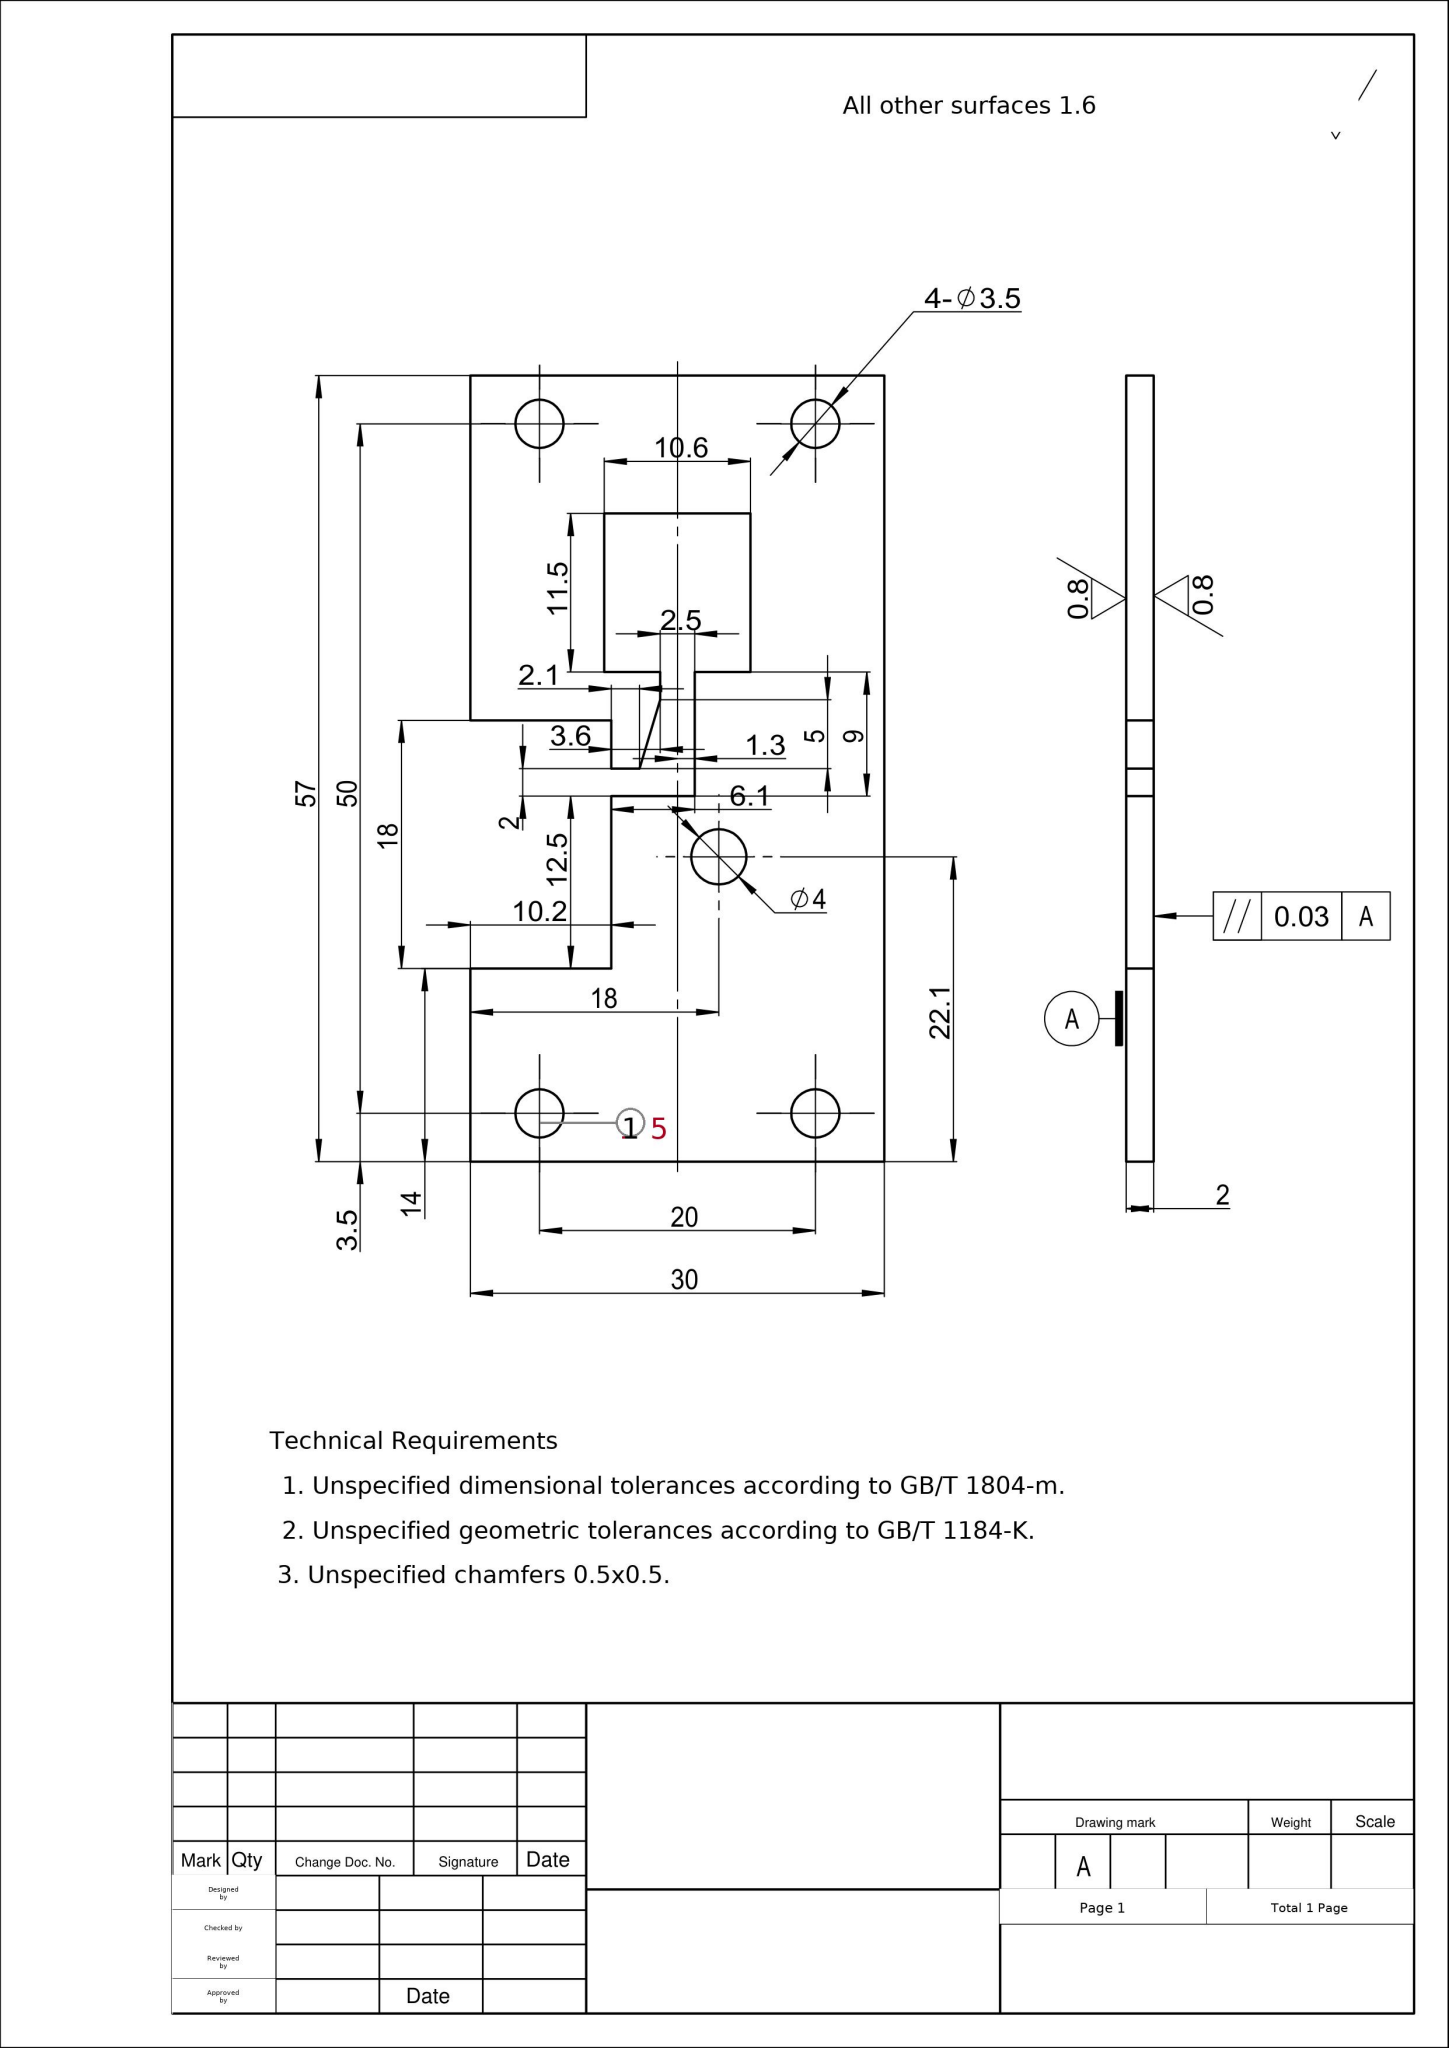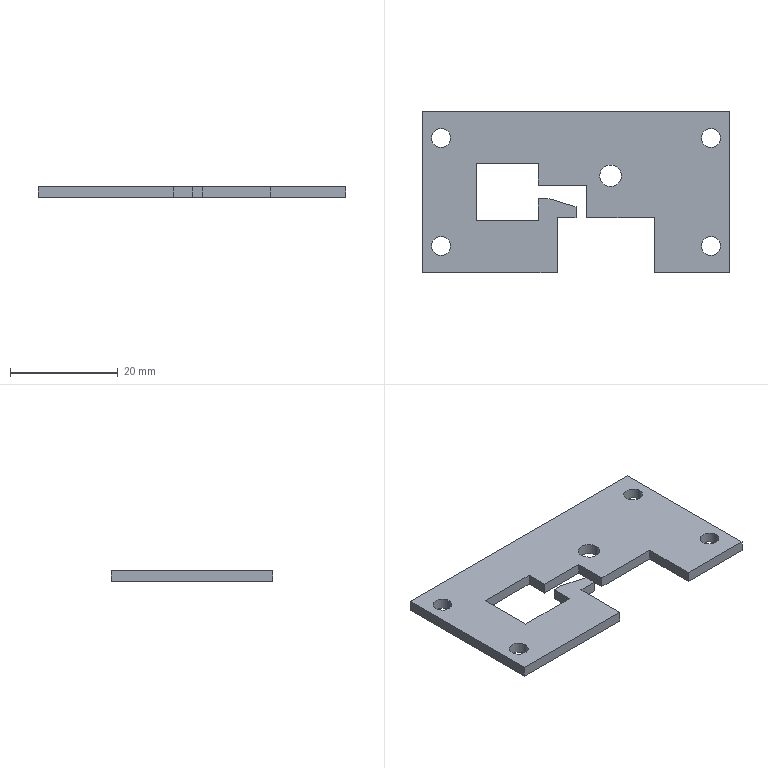Part | SolidWorks | mm | 1 solid | 31 faces | box 57 x 30 x 2 mm | volume 2640 mm3 | plane 21 | cylinder 10 | commonest cylinder face diameters 3.5 x8 4 x2
STEP:
#1=CARTESIAN_POINT('',(32.9,-12.,0.));
#2=VERTEX_POINT('',#1);
#3=CARTESIAN_POINT('',(36.9,-12.,0.));
#4=VERTEX_POINT('',#3);
#5=CARTESIAN_POINT('',(34.9,-12.,0.));
#6=DIRECTION('',(0.,0.,1.));
#7=DIRECTION('',(1.,0.,0.));
#8=AXIS2_PLACEMENT_3D('',#5,#6,#7);
#9=CIRCLE('',#8,2.);
#10=EDGE_CURVE('',#2,#4,#9,.T.);
#11=ORIENTED_EDGE('',*,*,#10,.F.);
#12=CARTESIAN_POINT('',(32.9,-12.,2.));
#13=VERTEX_POINT('',#12);
#14=CARTESIAN_POINT('',(32.9,-12.,0.));
#15=DIRECTION('',(0.,0.,1.));
#16=VECTOR('',#15,1000.);
#17=LINE('',#14,#16);
#18=EDGE_CURVE('',#2,#13,#17,.T.);
#19=ORIENTED_EDGE('',*,*,#18,.T.);
#20=CARTESIAN_POINT('',(36.9,-12.,2.));
#21=VERTEX_POINT('',#20);
#22=CARTESIAN_POINT('',(34.9,-12.,2.));
#23=DIRECTION('',(0.,0.,1.));
#24=DIRECTION('',(1.,0.,0.));
#25=AXIS2_PLACEMENT_3D('',#22,#23,#24);
#26=CIRCLE('',#25,2.);
#27=EDGE_CURVE('',#13,#21,#26,.T.);
#28=ORIENTED_EDGE('',*,*,#27,.T.);
#29=CARTESIAN_POINT('',(36.9,-12.,0.));
#30=DIRECTION('',(0.,0.,1.));
#31=VECTOR('',#30,1000.);
#32=LINE('',#29,#31);
#33=EDGE_CURVE('',#4,#21,#32,.T.);
#34=ORIENTED_EDGE('',*,*,#33,.F.);
#35=EDGE_LOOP('',(#11,#19,#28,#34));
#36=FACE_OUTER_BOUND('',#35,.T.);
#37=CARTESIAN_POINT('',(34.9,-12.,0.));
#38=DIRECTION('',(0.,0.,1.));
#39=DIRECTION('',(1.,0.,0.));
#40=AXIS2_PLACEMENT_3D('',#37,#38,#39);
#41=CYLINDRICAL_SURFACE('',#40,2.);
#42=ADVANCED_FACE('',(#36),#41,.F.);
#43=CARTESIAN_POINT('',(5.25,-25.,0.));
#44=VERTEX_POINT('',#43);
#45=CARTESIAN_POINT('',(1.75,-25.,0.));
#46=VERTEX_POINT('',#45);
#47=CARTESIAN_POINT('',(3.5,-25.,0.));
#48=DIRECTION('',(0.,0.,-1.));
#49=DIRECTION('',(1.,0.,0.));
#50=AXIS2_PLACEMENT_3D('',#47,#48,#49);
#51=CIRCLE('',#50,1.75);
#52=EDGE_CURVE('',#44,#46,#51,.T.);
#53=ORIENTED_EDGE('',*,*,#52,.T.);
#54=CARTESIAN_POINT('',(1.75,-25.,2.));
#55=VERTEX_POINT('',#54);
#56=CARTESIAN_POINT('',(1.75,-25.,-0.001));
#57=DIRECTION('',(0.,0.,1.));
#58=VECTOR('',#57,1000.);
#59=LINE('',#56,#58);
#60=EDGE_CURVE('',#46,#55,#59,.T.);
#61=ORIENTED_EDGE('',*,*,#60,.T.);
#62=CARTESIAN_POINT('',(5.25,-25.,2.));
#63=VERTEX_POINT('',#62);
#64=CARTESIAN_POINT('',(3.5,-25.,2.));
#65=DIRECTION('',(0.,0.,1.));
#66=DIRECTION('',(-1.,0.,0.));
#67=AXIS2_PLACEMENT_3D('',#64,#65,#66);
#68=CIRCLE('',#67,1.75);
#69=EDGE_CURVE('',#55,#63,#68,.T.);
#70=ORIENTED_EDGE('',*,*,#69,.T.);
#71=CARTESIAN_POINT('',(5.25,-25.,-0.001));
#72=DIRECTION('',(0.,0.,1.));
#73=VECTOR('',#72,1000.);
#74=LINE('',#71,#73);
#75=EDGE_CURVE('',#44,#63,#74,.T.);
#76=ORIENTED_EDGE('',*,*,#75,.F.);
#77=EDGE_LOOP('',(#53,#61,#70,#76));
#78=FACE_OUTER_BOUND('',#77,.T.);
#79=CARTESIAN_POINT('',(3.5,-25.,-0.001));
#80=DIRECTION('',(0.,0.,1.));
#81=DIRECTION('',(1.,0.,0.));
#82=AXIS2_PLACEMENT_3D('',#79,#80,#81);
#83=CYLINDRICAL_SURFACE('',#82,1.75);
#84=ADVANCED_FACE('',(#78),#83,.F.);
#85=CARTESIAN_POINT('',(55.25,-25.,0.));
#86=VERTEX_POINT('',#85);
#87=CARTESIAN_POINT('',(51.75,-25.,0.));
#88=VERTEX_POINT('',#87);
#89=CARTESIAN_POINT('',(53.5,-25.,0.));
#90=DIRECTION('',(0.,0.,-1.));
#91=DIRECTION('',(1.,0.,0.));
#92=AXIS2_PLACEMENT_3D('',#89,#90,#91);
#93=CIRCLE('',#92,1.75);
#94=EDGE_CURVE('',#86,#88,#93,.T.);
#95=ORIENTED_EDGE('',*,*,#94,.T.);
#96=CARTESIAN_POINT('',(51.75,-25.,2.));
#97=VERTEX_POINT('',#96);
#98=CARTESIAN_POINT('',(51.75,-25.,-0.001));
#99=DIRECTION('',(0.,0.,1.));
#100=VECTOR('',#99,1000.);
#101=LINE('',#98,#100);
#102=EDGE_CURVE('',#88,#97,#101,.T.);
#103=ORIENTED_EDGE('',*,*,#102,.T.);
#104=CARTESIAN_POINT('',(55.25,-25.,2.));
#105=VERTEX_POINT('',#104);
#106=CARTESIAN_POINT('',(53.5,-25.,2.));
#107=DIRECTION('',(0.,0.,1.));
#108=DIRECTION('',(-1.,0.,0.));
#109=AXIS2_PLACEMENT_3D('',#106,#107,#108);
#110=CIRCLE('',#109,1.75);
#111=EDGE_CURVE('',#97,#105,#110,.T.);
#112=ORIENTED_EDGE('',*,*,#111,.T.);
#113=CARTESIAN_POINT('',(55.25,-25.,-0.001));
#114=DIRECTION('',(0.,0.,1.));
#115=VECTOR('',#114,1000.);
#116=LINE('',#113,#115);
#117=EDGE_CURVE('',#86,#105,#116,.T.);
#118=ORIENTED_EDGE('',*,*,#117,.F.);
#119=EDGE_LOOP('',(#95,#103,#112,#118));
#120=FACE_OUTER_BOUND('',#119,.T.);
#121=CARTESIAN_POINT('',(53.5,-25.,-0.001));
#122=DIRECTION('',(0.,0.,1.));
#123=DIRECTION('',(1.,0.,0.));
#124=AXIS2_PLACEMENT_3D('',#121,#122,#123);
#125=CYLINDRICAL_SURFACE('',#124,1.75);
#126=ADVANCED_FACE('',(#120),#125,.F.);
#127=CARTESIAN_POINT('',(55.25,-5.,0.));
#128=VERTEX_POINT('',#127);
#129=CARTESIAN_POINT('',(51.75,-5.,0.));
#130=VERTEX_POINT('',#129);
#131=CARTESIAN_POINT('',(53.5,-5.,0.));
#132=DIRECTION('',(0.,0.,-1.));
#133=DIRECTION('',(1.,0.,0.));
#134=AXIS2_PLACEMENT_3D('',#131,#132,#133);
#135=CIRCLE('',#134,1.75);
#136=EDGE_CURVE('',#128,#130,#135,.T.);
#137=ORIENTED_EDGE('',*,*,#136,.T.);
#138=CARTESIAN_POINT('',(51.75,-5.,2.));
#139=VERTEX_POINT('',#138);
#140=CARTESIAN_POINT('',(51.75,-5.,-0.001));
#141=DIRECTION('',(0.,0.,1.));
#142=VECTOR('',#141,1000.);
#143=LINE('',#140,#142);
#144=EDGE_CURVE('',#130,#139,#143,.T.);
#145=ORIENTED_EDGE('',*,*,#144,.T.);
#146=CARTESIAN_POINT('',(55.25,-5.,2.));
#147=VERTEX_POINT('',#146);
#148=CARTESIAN_POINT('',(53.5,-5.,2.));
#149=DIRECTION('',(0.,0.,1.));
#150=DIRECTION('',(1.,0.,0.));
#151=AXIS2_PLACEMENT_3D('',#148,#149,#150);
#152=CIRCLE('',#151,1.75);
#153=EDGE_CURVE('',#139,#147,#152,.T.);
#154=ORIENTED_EDGE('',*,*,#153,.T.);
#155=CARTESIAN_POINT('',(55.25,-5.,-0.001));
#156=DIRECTION('',(0.,0.,1.));
#157=VECTOR('',#156,1000.);
#158=LINE('',#155,#157);
#159=EDGE_CURVE('',#128,#147,#158,.T.);
#160=ORIENTED_EDGE('',*,*,#159,.F.);
#161=EDGE_LOOP('',(#137,#145,#154,#160));
#162=FACE_OUTER_BOUND('',#161,.T.);
#163=CARTESIAN_POINT('',(53.5,-5.,-0.001));
#164=DIRECTION('',(0.,0.,1.));
#165=DIRECTION('',(1.,0.,0.));
#166=AXIS2_PLACEMENT_3D('',#163,#164,#165);
#167=CYLINDRICAL_SURFACE('',#166,1.75);
#168=ADVANCED_FACE('',(#162),#167,.F.);
#169=CARTESIAN_POINT('',(5.25,-5.,0.));
#170=VERTEX_POINT('',#169);
#171=CARTESIAN_POINT('',(1.75,-5.,0.));
#172=VERTEX_POINT('',#171);
#173=CARTESIAN_POINT('',(3.5,-5.,0.));
#174=DIRECTION('',(0.,0.,-1.));
#175=DIRECTION('',(1.,0.,0.));
#176=AXIS2_PLACEMENT_3D('',#173,#174,#175);
#177=CIRCLE('',#176,1.75);
#178=EDGE_CURVE('',#170,#172,#177,.T.);
#179=ORIENTED_EDGE('',*,*,#178,.T.);
#180=CARTESIAN_POINT('',(1.75,-5.,2.));
#181=VERTEX_POINT('',#180);
#182=CARTESIAN_POINT('',(1.75,-5.,-0.001));
#183=DIRECTION('',(0.,0.,1.));
#184=VECTOR('',#183,1000.);
#185=LINE('',#182,#184);
#186=EDGE_CURVE('',#172,#181,#185,.T.);
#187=ORIENTED_EDGE('',*,*,#186,.T.);
#188=CARTESIAN_POINT('',(5.25,-5.,2.));
#189=VERTEX_POINT('',#188);
#190=CARTESIAN_POINT('',(3.5,-5.,2.));
#191=DIRECTION('',(0.,0.,1.));
#192=DIRECTION('',(1.,0.,0.));
#193=AXIS2_PLACEMENT_3D('',#190,#191,#192);
#194=CIRCLE('',#193,1.75);
#195=EDGE_CURVE('',#181,#189,#194,.T.);
#196=ORIENTED_EDGE('',*,*,#195,.T.);
#197=CARTESIAN_POINT('',(5.25,-5.,-0.001));
#198=DIRECTION('',(0.,0.,1.));
#199=VECTOR('',#198,1000.);
#200=LINE('',#197,#199);
#201=EDGE_CURVE('',#170,#189,#200,.T.);
#202=ORIENTED_EDGE('',*,*,#201,.F.);
#203=EDGE_LOOP('',(#179,#187,#196,#202));
#204=FACE_OUTER_BOUND('',#203,.T.);
#205=CARTESIAN_POINT('',(3.5,-5.,-0.001));
#206=DIRECTION('',(0.,0.,1.));
#207=DIRECTION('',(1.,0.,0.));
#208=AXIS2_PLACEMENT_3D('',#205,#206,#207);
#209=CYLINDRICAL_SURFACE('',#208,1.75);
#210=ADVANCED_FACE('',(#204),#209,.F.);
#211=CARTESIAN_POINT('',(43.,-19.8,2.));
#212=VERTEX_POINT('',#211);
#213=CARTESIAN_POINT('',(30.5,-19.8,2.));
#214=VERTEX_POINT('',#213);
#215=CARTESIAN_POINT('',(25.,-19.8,2.));
#216=DIRECTION('',(-1.,0.,0.));
#217=VECTOR('',#216,1000.);
#218=LINE('',#215,#217);
#219=EDGE_CURVE('',#212,#214,#218,.T.);
#220=ORIENTED_EDGE('',*,*,#219,.T.);
#221=CARTESIAN_POINT('',(30.5,-19.8,0.));
#222=VERTEX_POINT('',#221);
#223=CARTESIAN_POINT('',(30.5,-19.8,-0.001));
#224=DIRECTION('',(0.,0.,-1.));
#225=VECTOR('',#224,1000.);
#226=LINE('',#223,#225);
#227=EDGE_CURVE('',#214,#222,#226,.T.);
#228=ORIENTED_EDGE('',*,*,#227,.T.);
#229=CARTESIAN_POINT('',(43.,-19.8,0.));
#230=VERTEX_POINT('',#229);
#231=CARTESIAN_POINT('',(25.,-19.8,0.));
#232=DIRECTION('',(1.,0.,0.));
#233=VECTOR('',#232,1000.);
#234=LINE('',#231,#233);
#235=EDGE_CURVE('',#222,#230,#234,.T.);
#236=ORIENTED_EDGE('',*,*,#235,.T.);
#237=CARTESIAN_POINT('',(43.,-19.8,-0.001));
#238=DIRECTION('',(0.,0.,1.));
#239=VECTOR('',#238,1000.);
#240=LINE('',#237,#239);
#241=EDGE_CURVE('',#230,#212,#240,.T.);
#242=ORIENTED_EDGE('',*,*,#241,.T.);
#243=EDGE_LOOP('',(#220,#228,#236,#242));
#244=FACE_OUTER_BOUND('',#243,.T.);
#245=CARTESIAN_POINT('',(25.,-19.8,-0.001));
#246=DIRECTION('',(0.,1.,0.));
#247=DIRECTION('',(0.,0.,1.));
#248=AXIS2_PLACEMENT_3D('',#245,#246,#247);
#249=PLANE('',#248);
#250=ADVANCED_FACE('',(#244),#249,.F.);
#251=CARTESIAN_POINT('',(0.,-30.,0.));
#252=VERTEX_POINT('',#251);
#253=CARTESIAN_POINT('',(25.,-30.,0.));
#254=VERTEX_POINT('',#253);
#255=CARTESIAN_POINT('',(0.,-30.,0.));
#256=DIRECTION('',(1.,0.,0.));
#257=VECTOR('',#256,1000.);
#258=LINE('',#255,#257);
#259=EDGE_CURVE('',#252,#254,#258,.T.);
#260=ORIENTED_EDGE('',*,*,#259,.T.);
#261=CARTESIAN_POINT('',(25.,-30.,2.));
#262=VERTEX_POINT('',#261);
#263=CARTESIAN_POINT('',(25.,-30.,-0.001));
#264=DIRECTION('',(0.,0.,1.));
#265=VECTOR('',#264,1000.);
#266=LINE('',#263,#265);
#267=EDGE_CURVE('',#254,#262,#266,.T.);
#268=ORIENTED_EDGE('',*,*,#267,.T.);
#269=CARTESIAN_POINT('',(0.,-30.,2.));
#270=VERTEX_POINT('',#269);
#271=CARTESIAN_POINT('',(0.,-30.,2.));
#272=DIRECTION('',(1.,0.,0.));
#273=VECTOR('',#272,1000.);
#274=LINE('',#271,#273);
#275=EDGE_CURVE('',#270,#262,#274,.T.);
#276=ORIENTED_EDGE('',*,*,#275,.F.);
#277=CARTESIAN_POINT('',(0.,-30.,2.));
#278=DIRECTION('',(0.,0.,-1.));
#279=VECTOR('',#278,1000.);
#280=LINE('',#277,#279);
#281=EDGE_CURVE('',#270,#252,#280,.T.);
#282=ORIENTED_EDGE('',*,*,#281,.T.);
#283=EDGE_LOOP('',(#260,#268,#276,#282));
#284=FACE_OUTER_BOUND('',#283,.T.);
#285=CARTESIAN_POINT('',(0.,-30.,2.));
#286=DIRECTION('',(0.,1.,0.));
#287=DIRECTION('',(0.,0.,1.));
#288=AXIS2_PLACEMENT_3D('',#285,#286,#287);
#289=PLANE('',#288);
#290=ADVANCED_FACE('',(#284),#289,.F.);
#291=CARTESIAN_POINT('',(0.,0.,0.));
#292=VERTEX_POINT('',#291);
#293=CARTESIAN_POINT('',(0.,0.,0.));
#294=DIRECTION('',(0.,-1.,0.));
#295=VECTOR('',#294,1000.);
#296=LINE('',#293,#295);
#297=EDGE_CURVE('',#292,#252,#296,.T.);
#298=ORIENTED_EDGE('',*,*,#297,.T.);
#299=ORIENTED_EDGE('',*,*,#281,.F.);
#300=CARTESIAN_POINT('',(0.,0.,2.));
#301=VERTEX_POINT('',#300);
#302=CARTESIAN_POINT('',(0.,0.,2.));
#303=DIRECTION('',(0.,-1.,0.));
#304=VECTOR('',#303,1000.);
#305=LINE('',#302,#304);
#306=EDGE_CURVE('',#301,#270,#305,.T.);
#307=ORIENTED_EDGE('',*,*,#306,.F.);
#308=CARTESIAN_POINT('',(0.,0.,2.));
#309=DIRECTION('',(0.,0.,-1.));
#310=VECTOR('',#309,1000.);
#311=LINE('',#308,#310);
#312=EDGE_CURVE('',#301,#292,#311,.T.);
#313=ORIENTED_EDGE('',*,*,#312,.T.);
#314=EDGE_LOOP('',(#298,#299,#307,#313));
#315=FACE_OUTER_BOUND('',#314,.T.);
#316=CARTESIAN_POINT('',(0.,0.,2.));
#317=DIRECTION('',(1.,0.,0.));
#318=DIRECTION('',(-0.,1.,0.));
#319=AXIS2_PLACEMENT_3D('',#316,#317,#318);
#320=PLANE('',#319);
#321=ADVANCED_FACE('',(#315),#320,.F.);
#322=CARTESIAN_POINT('',(43.,-30.,2.));
#323=VERTEX_POINT('',#322);
#324=CARTESIAN_POINT('',(57.,-30.,2.));
#325=VERTEX_POINT('',#324);
#326=CARTESIAN_POINT('',(0.,-30.,2.));
#327=DIRECTION('',(1.,0.,0.));
#328=VECTOR('',#327,1000.);
#329=LINE('',#326,#328);
#330=EDGE_CURVE('',#323,#325,#329,.T.);
#331=ORIENTED_EDGE('',*,*,#330,.F.);
#332=CARTESIAN_POINT('',(43.,-30.,0.));
#333=VERTEX_POINT('',#332);
#334=CARTESIAN_POINT('',(43.,-30.,-0.001));
#335=DIRECTION('',(0.,0.,1.));
#336=VECTOR('',#335,1000.);
#337=LINE('',#334,#336);
#338=EDGE_CURVE('',#333,#323,#337,.T.);
#339=ORIENTED_EDGE('',*,*,#338,.F.);
#340=CARTESIAN_POINT('',(57.,-30.,0.));
#341=VERTEX_POINT('',#340);
#342=CARTESIAN_POINT('',(0.,-30.,0.));
#343=DIRECTION('',(1.,0.,0.));
#344=VECTOR('',#343,1000.);
#345=LINE('',#342,#344);
#346=EDGE_CURVE('',#333,#341,#345,.T.);
#347=ORIENTED_EDGE('',*,*,#346,.T.);
#348=CARTESIAN_POINT('',(57.,-30.,2.));
#349=DIRECTION('',(0.,0.,-1.));
#350=VECTOR('',#349,1000.);
#351=LINE('',#348,#350);
#352=EDGE_CURVE('',#325,#341,#351,.T.);
#353=ORIENTED_EDGE('',*,*,#352,.F.);
#354=EDGE_LOOP('',(#331,#339,#347,#353));
#355=FACE_OUTER_BOUND('',#354,.T.);
#356=CARTESIAN_POINT('',(0.,-30.,2.));
#357=DIRECTION('',(0.,1.,0.));
#358=DIRECTION('',(0.,0.,1.));
#359=AXIS2_PLACEMENT_3D('',#356,#357,#358);
#360=PLANE('',#359);
#361=ADVANCED_FACE('',(#355),#360,.F.);
#362=CARTESIAN_POINT('',(57.,0.,0.));
#363=VERTEX_POINT('',#362);
#364=CARTESIAN_POINT('',(57.,0.,0.));
#365=DIRECTION('',(-0.,1.,0.));
#366=VECTOR('',#365,1000.);
#367=LINE('',#364,#366);
#368=EDGE_CURVE('',#341,#363,#367,.T.);
#369=ORIENTED_EDGE('',*,*,#368,.T.);
#370=CARTESIAN_POINT('',(57.,0.,2.));
#371=VERTEX_POINT('',#370);
#372=CARTESIAN_POINT('',(57.,0.,2.));
#373=DIRECTION('',(0.,0.,-1.));
#374=VECTOR('',#373,1000.);
#375=LINE('',#372,#374);
#376=EDGE_CURVE('',#371,#363,#375,.T.);
#377=ORIENTED_EDGE('',*,*,#376,.F.);
#378=CARTESIAN_POINT('',(57.,0.,2.));
#379=DIRECTION('',(-0.,1.,0.));
#380=VECTOR('',#379,1000.);
#381=LINE('',#378,#380);
#382=EDGE_CURVE('',#325,#371,#381,.T.);
#383=ORIENTED_EDGE('',*,*,#382,.F.);
#384=ORIENTED_EDGE('',*,*,#352,.T.);
#385=EDGE_LOOP('',(#369,#377,#383,#384));
#386=FACE_OUTER_BOUND('',#385,.T.);
#387=CARTESIAN_POINT('',(57.,0.,2.));
#388=DIRECTION('',(-1.,-0.,0.));
#389=DIRECTION('',(0.,-1.,0.));
#390=AXIS2_PLACEMENT_3D('',#387,#388,#389);
#391=PLANE('',#390);
#392=ADVANCED_FACE('',(#386),#391,.F.);
#393=CARTESIAN_POINT('',(0.,0.,0.));
#394=DIRECTION('',(-1.,0.,0.));
#395=VECTOR('',#394,1000.);
#396=LINE('',#393,#395);
#397=EDGE_CURVE('',#363,#292,#396,.T.);
#398=ORIENTED_EDGE('',*,*,#397,.T.);
#399=ORIENTED_EDGE('',*,*,#312,.F.);
#400=CARTESIAN_POINT('',(0.,0.,2.));
#401=DIRECTION('',(-1.,0.,0.));
#402=VECTOR('',#401,1000.);
#403=LINE('',#400,#402);
#404=EDGE_CURVE('',#371,#301,#403,.T.);
#405=ORIENTED_EDGE('',*,*,#404,.F.);
#406=ORIENTED_EDGE('',*,*,#376,.T.);
#407=EDGE_LOOP('',(#398,#399,#405,#406));
#408=FACE_OUTER_BOUND('',#407,.T.);
#409=CARTESIAN_POINT('',(0.,0.,2.));
#410=DIRECTION('',(0.,-1.,0.));
#411=DIRECTION('',(0.,0.,-1.));
#412=AXIS2_PLACEMENT_3D('',#409,#410,#411);
#413=PLANE('',#412);
#414=ADVANCED_FACE('',(#408),#413,.F.);
#415=CARTESIAN_POINT('',(34.9,-12.,2.));
#416=DIRECTION('',(0.,0.,1.));
#417=DIRECTION('',(1.,0.,0.));
#418=AXIS2_PLACEMENT_3D('',#415,#416,#417);
#419=CIRCLE('',#418,2.);
#420=EDGE_CURVE('',#21,#13,#419,.T.);
#421=ORIENTED_EDGE('',*,*,#420,.F.);
#422=ORIENTED_EDGE('',*,*,#27,.F.);
#423=EDGE_LOOP('',(#421,#422));
#424=FACE_BOUND('',#423,.T.);
#425=CARTESIAN_POINT('',(30.5,-13.75,2.));
#426=VERTEX_POINT('',#425);
#427=CARTESIAN_POINT('',(30.5,-19.874,2.));
#428=DIRECTION('',(0.,1.,0.));
#429=VECTOR('',#428,1000.);
#430=LINE('',#427,#429);
#431=EDGE_CURVE('',#214,#426,#430,.T.);
#432=ORIENTED_EDGE('',*,*,#431,.F.);
#433=ORIENTED_EDGE('',*,*,#219,.F.);
#434=CARTESIAN_POINT('',(43.,-19.8,2.));
#435=DIRECTION('',(0.,1.,0.));
#436=VECTOR('',#435,1000.);
#437=LINE('',#434,#436);
#438=EDGE_CURVE('',#323,#212,#437,.T.);
#439=ORIENTED_EDGE('',*,*,#438,.F.);
#440=ORIENTED_EDGE('',*,*,#330,.T.);
#441=ORIENTED_EDGE('',*,*,#382,.T.);
#442=ORIENTED_EDGE('',*,*,#404,.T.);
#443=ORIENTED_EDGE('',*,*,#306,.T.);
#444=ORIENTED_EDGE('',*,*,#275,.T.);
#445=CARTESIAN_POINT('',(25.,-19.8,2.));
#446=VERTEX_POINT('',#445);
#447=CARTESIAN_POINT('',(25.,-19.8,2.));
#448=DIRECTION('',(0.,-1.,0.));
#449=VECTOR('',#448,1000.);
#450=LINE('',#447,#449);
#451=EDGE_CURVE('',#446,#262,#450,.T.);
#452=ORIENTED_EDGE('',*,*,#451,.F.);
#453=CARTESIAN_POINT('',(28.5,-19.8,2.));
#454=VERTEX_POINT('',#453);
#455=CARTESIAN_POINT('',(25.,-19.8,2.));
#456=DIRECTION('',(-1.,0.,0.));
#457=VECTOR('',#456,1000.);
#458=LINE('',#455,#457);
#459=EDGE_CURVE('',#454,#446,#458,.T.);
#460=ORIENTED_EDGE('',*,*,#459,.F.);
#461=CARTESIAN_POINT('',(28.5,-17.75,2.));
#462=VERTEX_POINT('',#461);
#463=CARTESIAN_POINT('',(28.5,-19.874,2.));
#464=DIRECTION('',(0.,-1.,0.));
#465=VECTOR('',#464,1000.);
#466=LINE('',#463,#465);
#467=EDGE_CURVE('',#462,#454,#466,.T.);
#468=ORIENTED_EDGE('',*,*,#467,.F.);
#469=CARTESIAN_POINT('',(23.5,-16.25,2.));
#470=VERTEX_POINT('',#469);
#471=CARTESIAN_POINT('',(28.5,-17.75,2.));
#472=DIRECTION('',(0.9578,-0.2873,0.));
#473=VECTOR('',#472,1000.);
#474=LINE('',#471,#473);
#475=EDGE_CURVE('',#470,#462,#474,.T.);
#476=ORIENTED_EDGE('',*,*,#475,.F.);
#477=CARTESIAN_POINT('',(21.5,-16.25,2.));
#478=VERTEX_POINT('',#477);
#479=CARTESIAN_POINT('',(21.5,-16.25,2.));
#480=DIRECTION('',(1.,0.,0.));
#481=VECTOR('',#480,1000.);
#482=LINE('',#479,#481);
#483=EDGE_CURVE('',#478,#470,#482,.T.);
#484=ORIENTED_EDGE('',*,*,#483,.F.);
#485=CARTESIAN_POINT('',(21.5,-20.3,2.));
#486=VERTEX_POINT('',#485);
#487=CARTESIAN_POINT('',(21.5,-16.25,2.));
#488=DIRECTION('',(0.,1.,0.));
#489=VECTOR('',#488,1000.);
#490=LINE('',#487,#489);
#491=EDGE_CURVE('',#486,#478,#490,.T.);
#492=ORIENTED_EDGE('',*,*,#491,.F.);
#493=CARTESIAN_POINT('',(10.,-20.3,2.));
#494=VERTEX_POINT('',#493);
#495=CARTESIAN_POINT('',(10.,-20.3,2.));
#496=DIRECTION('',(1.,0.,0.));
#497=VECTOR('',#496,1000.);
#498=LINE('',#495,#497);
#499=EDGE_CURVE('',#494,#486,#498,.T.);
#500=ORIENTED_EDGE('',*,*,#499,.F.);
#501=CARTESIAN_POINT('',(10.,-9.7,2.));
#502=VERTEX_POINT('',#501);
#503=CARTESIAN_POINT('',(10.,-9.7,2.));
#504=DIRECTION('',(0.,-1.,0.));
#505=VECTOR('',#504,1000.);
#506=LINE('',#503,#505);
#507=EDGE_CURVE('',#502,#494,#506,.T.);
#508=ORIENTED_EDGE('',*,*,#507,.F.);
#509=CARTESIAN_POINT('',(21.5,-9.7,2.));
#510=VERTEX_POINT('',#509);
#511=CARTESIAN_POINT('',(10.,-9.7,2.));
#512=DIRECTION('',(-1.,0.,0.));
#513=VECTOR('',#512,1000.);
#514=LINE('',#511,#513);
#515=EDGE_CURVE('',#510,#502,#514,.T.);
#516=ORIENTED_EDGE('',*,*,#515,.F.);
#517=CARTESIAN_POINT('',(21.5,-13.75,2.));
#518=VERTEX_POINT('',#517);
#519=CARTESIAN_POINT('',(21.5,-9.7,2.));
#520=DIRECTION('',(0.,1.,0.));
#521=VECTOR('',#520,1000.);
#522=LINE('',#519,#521);
#523=EDGE_CURVE('',#518,#510,#522,.T.);
#524=ORIENTED_EDGE('',*,*,#523,.F.);
#525=CARTESIAN_POINT('',(21.5,-13.75,2.));
#526=DIRECTION('',(-1.,0.,0.));
#527=VECTOR('',#526,1000.);
#528=LINE('',#525,#527);
#529=EDGE_CURVE('',#426,#518,#528,.T.);
#530=ORIENTED_EDGE('',*,*,#529,.F.);
#531=EDGE_LOOP('',(#432,#433,#439,#440,#441,#442,#443,#444,#452,#460,#468,#476,#484,#492,#500,#508,#516,#524,#530));
#532=FACE_OUTER_BOUND('',#531,.T.);
#533=CARTESIAN_POINT('',(3.5,-25.,2.));
#534=DIRECTION('',(0.,0.,1.));
#535=DIRECTION('',(-1.,0.,0.));
#536=AXIS2_PLACEMENT_3D('',#533,#534,#535);
#537=CIRCLE('',#536,1.75);
#538=EDGE_CURVE('',#63,#55,#537,.T.);
#539=ORIENTED_EDGE('',*,*,#538,.F.);
#540=ORIENTED_EDGE('',*,*,#69,.F.);
#541=EDGE_LOOP('',(#539,#540));
#542=FACE_BOUND('',#541,.T.);
#543=CARTESIAN_POINT('',(53.5,-25.,2.));
#544=DIRECTION('',(0.,0.,1.));
#545=DIRECTION('',(-1.,0.,0.));
#546=AXIS2_PLACEMENT_3D('',#543,#544,#545);
#547=CIRCLE('',#546,1.75);
#548=EDGE_CURVE('',#105,#97,#547,.T.);
#549=ORIENTED_EDGE('',*,*,#548,.F.);
#550=ORIENTED_EDGE('',*,*,#111,.F.);
#551=EDGE_LOOP('',(#549,#550));
#552=FACE_BOUND('',#551,.T.);
#553=CARTESIAN_POINT('',(53.5,-5.,2.));
#554=DIRECTION('',(0.,0.,1.));
#555=DIRECTION('',(1.,0.,0.));
#556=AXIS2_PLACEMENT_3D('',#553,#554,#555);
#557=CIRCLE('',#556,1.75);
#558=EDGE_CURVE('',#147,#139,#557,.T.);
#559=ORIENTED_EDGE('',*,*,#558,.F.);
#560=ORIENTED_EDGE('',*,*,#153,.F.);
#561=EDGE_LOOP('',(#559,#560));
#562=FACE_BOUND('',#561,.T.);
#563=CARTESIAN_POINT('',(3.5,-5.,2.));
#564=DIRECTION('',(0.,0.,1.));
#565=DIRECTION('',(1.,0.,0.));
#566=AXIS2_PLACEMENT_3D('',#563,#564,#565);
#567=CIRCLE('',#566,1.75);
#568=EDGE_CURVE('',#189,#181,#567,.T.);
#569=ORIENTED_EDGE('',*,*,#568,.F.);
#570=ORIENTED_EDGE('',*,*,#195,.F.);
#571=EDGE_LOOP('',(#569,#570));
#572=FACE_BOUND('',#571,.T.);
#573=CARTESIAN_POINT('',(0.,-30.,2.));
#574=DIRECTION('',(0.,0.,1.));
#575=DIRECTION('',(1.,0.,0.));
#576=AXIS2_PLACEMENT_3D('',#573,#574,#575);
#577=PLANE('',#576);
#578=ADVANCED_FACE('',(#424,#532,#542,#552,#562,#572),#577,.T.);
#579=CARTESIAN_POINT('',(34.9,-12.,0.));
#580=DIRECTION('',(0.,0.,1.));
#581=DIRECTION('',(1.,0.,0.));
#582=AXIS2_PLACEMENT_3D('',#579,#580,#581);
#583=CIRCLE('',#582,2.);
#584=EDGE_CURVE('',#4,#2,#583,.T.);
#585=ORIENTED_EDGE('',*,*,#584,.T.);
#586=ORIENTED_EDGE('',*,*,#10,.T.);
#587=EDGE_LOOP('',(#585,#586));
#588=FACE_BOUND('',#587,.T.);
#589=ORIENTED_EDGE('',*,*,#235,.F.);
#590=CARTESIAN_POINT('',(30.5,-13.75,0.));
#591=VERTEX_POINT('',#590);
#592=CARTESIAN_POINT('',(30.5,-19.874,0.));
#593=DIRECTION('',(0.,1.,0.));
#594=VECTOR('',#593,1000.);
#595=LINE('',#592,#594);
#596=EDGE_CURVE('',#222,#591,#595,.T.);
#597=ORIENTED_EDGE('',*,*,#596,.T.);
#598=CARTESIAN_POINT('',(21.5,-13.75,0.));
#599=VERTEX_POINT('',#598);
#600=CARTESIAN_POINT('',(28.5,-13.75,0.));
#601=DIRECTION('',(-1.,-0.,0.));
#602=VECTOR('',#601,1000.);
#603=LINE('',#600,#602);
#604=EDGE_CURVE('',#591,#599,#603,.T.);
#605=ORIENTED_EDGE('',*,*,#604,.T.);
#606=CARTESIAN_POINT('',(21.5,-9.7,0.));
#607=VERTEX_POINT('',#606);
#608=CARTESIAN_POINT('',(21.5,-9.7,0.));
#609=DIRECTION('',(0.,1.,0.));
#610=VECTOR('',#609,1000.);
#611=LINE('',#608,#610);
#612=EDGE_CURVE('',#599,#607,#611,.T.);
#613=ORIENTED_EDGE('',*,*,#612,.T.);
#614=CARTESIAN_POINT('',(10.,-9.7,0.));
#615=VERTEX_POINT('',#614);
#616=CARTESIAN_POINT('',(10.,-9.7,0.));
#617=DIRECTION('',(-1.,0.,0.));
#618=VECTOR('',#617,1000.);
#619=LINE('',#616,#618);
#620=EDGE_CURVE('',#607,#615,#619,.T.);
#621=ORIENTED_EDGE('',*,*,#620,.T.);
#622=CARTESIAN_POINT('',(10.,-20.3,0.));
#623=VERTEX_POINT('',#622);
#624=CARTESIAN_POINT('',(10.,-9.7,0.));
#625=DIRECTION('',(0.,-1.,0.));
#626=VECTOR('',#625,1000.);
#627=LINE('',#624,#626);
#628=EDGE_CURVE('',#615,#623,#627,.T.);
#629=ORIENTED_EDGE('',*,*,#628,.T.);
#630=CARTESIAN_POINT('',(21.5,-20.3,0.));
#631=VERTEX_POINT('',#630);
#632=CARTESIAN_POINT('',(10.,-20.3,0.));
#633=DIRECTION('',(1.,0.,0.));
#634=VECTOR('',#633,1000.);
#635=LINE('',#632,#634);
#636=EDGE_CURVE('',#623,#631,#635,.T.);
#637=ORIENTED_EDGE('',*,*,#636,.T.);
#638=CARTESIAN_POINT('',(21.5,-16.25,0.));
#639=VERTEX_POINT('',#638);
#640=CARTESIAN_POINT('',(21.5,-16.25,0.));
#641=DIRECTION('',(0.,1.,0.));
#642=VECTOR('',#641,1000.);
#643=LINE('',#640,#642);
#644=EDGE_CURVE('',#631,#639,#643,.T.);
#645=ORIENTED_EDGE('',*,*,#644,.T.);
#646=CARTESIAN_POINT('',(23.5,-16.25,0.));
#647=VERTEX_POINT('',#646);
#648=CARTESIAN_POINT('',(21.5,-16.25,0.));
#649=DIRECTION('',(1.,0.,0.));
#650=VECTOR('',#649,1000.);
#651=LINE('',#648,#650);
#652=EDGE_CURVE('',#639,#647,#651,.T.);
#653=ORIENTED_EDGE('',*,*,#652,.T.);
#654=CARTESIAN_POINT('',(28.5,-17.75,0.));
#655=VERTEX_POINT('',#654);
#656=CARTESIAN_POINT('',(28.5,-17.75,0.));
#657=DIRECTION('',(0.9578,-0.2873,0.));
#658=VECTOR('',#657,1000.);
#659=LINE('',#656,#658);
#660=EDGE_CURVE('',#647,#655,#659,.T.);
#661=ORIENTED_EDGE('',*,*,#660,.T.);
#662=CARTESIAN_POINT('',(28.5,-19.8,0.));
#663=VERTEX_POINT('',#662);
#664=CARTESIAN_POINT('',(28.5,-19.874,0.));
#665=DIRECTION('',(0.,-1.,0.));
#666=VECTOR('',#665,1000.);
#667=LINE('',#664,#666);
#668=EDGE_CURVE('',#655,#663,#667,.T.);
#669=ORIENTED_EDGE('',*,*,#668,.T.);
#670=CARTESIAN_POINT('',(25.,-19.8,0.));
#671=VERTEX_POINT('',#670);
#672=CARTESIAN_POINT('',(25.,-19.8,0.));
#673=DIRECTION('',(1.,0.,0.));
#674=VECTOR('',#673,1000.);
#675=LINE('',#672,#674);
#676=EDGE_CURVE('',#671,#663,#675,.T.);
#677=ORIENTED_EDGE('',*,*,#676,.F.);
#678=CARTESIAN_POINT('',(25.,-19.8,0.));
#679=DIRECTION('',(0.,1.,0.));
#680=VECTOR('',#679,1000.);
#681=LINE('',#678,#680);
#682=EDGE_CURVE('',#254,#671,#681,.T.);
#683=ORIENTED_EDGE('',*,*,#682,.F.);
#684=ORIENTED_EDGE('',*,*,#259,.F.);
#685=ORIENTED_EDGE('',*,*,#297,.F.);
#686=ORIENTED_EDGE('',*,*,#397,.F.);
#687=ORIENTED_EDGE('',*,*,#368,.F.);
#688=ORIENTED_EDGE('',*,*,#346,.F.);
#689=CARTESIAN_POINT('',(43.,-19.8,0.));
#690=DIRECTION('',(0.,-1.,0.));
#691=VECTOR('',#690,1000.);
#692=LINE('',#689,#691);
#693=EDGE_CURVE('',#230,#333,#692,.T.);
#694=ORIENTED_EDGE('',*,*,#693,.F.);
#695=EDGE_LOOP('',(#589,#597,#605,#613,#621,#629,#637,#645,#653,#661,#669,#677,#683,#684,#685,#686,#687,#688,#694));
#696=FACE_OUTER_BOUND('',#695,.T.);
#697=ORIENTED_EDGE('',*,*,#52,.F.);
#698=CARTESIAN_POINT('',(3.5,-25.,0.));
#699=DIRECTION('',(0.,0.,-1.));
#700=DIRECTION('',(1.,0.,0.));
#701=AXIS2_PLACEMENT_3D('',#698,#699,#700);
#702=CIRCLE('',#701,1.75);
#703=EDGE_CURVE('',#46,#44,#702,.T.);
#704=ORIENTED_EDGE('',*,*,#703,.F.);
#705=EDGE_LOOP('',(#697,#704));
#706=FACE_BOUND('',#705,.T.);
#707=ORIENTED_EDGE('',*,*,#94,.F.);
#708=CARTESIAN_POINT('',(53.5,-25.,0.));
#709=DIRECTION('',(0.,0.,-1.));
#710=DIRECTION('',(1.,0.,0.));
#711=AXIS2_PLACEMENT_3D('',#708,#709,#710);
#712=CIRCLE('',#711,1.75);
#713=EDGE_CURVE('',#88,#86,#712,.T.);
#714=ORIENTED_EDGE('',*,*,#713,.F.);
#715=EDGE_LOOP('',(#707,#714));
#716=FACE_BOUND('',#715,.T.);
#717=ORIENTED_EDGE('',*,*,#136,.F.);
#718=CARTESIAN_POINT('',(53.5,-5.,0.));
#719=DIRECTION('',(0.,0.,-1.));
#720=DIRECTION('',(1.,0.,0.));
#721=AXIS2_PLACEMENT_3D('',#718,#719,#720);
#722=CIRCLE('',#721,1.75);
#723=EDGE_CURVE('',#130,#128,#722,.T.);
#724=ORIENTED_EDGE('',*,*,#723,.F.);
#725=EDGE_LOOP('',(#717,#724));
#726=FACE_BOUND('',#725,.T.);
#727=ORIENTED_EDGE('',*,*,#178,.F.);
#728=CARTESIAN_POINT('',(3.5,-5.,0.));
#729=DIRECTION('',(0.,0.,-1.));
#730=DIRECTION('',(1.,0.,0.));
#731=AXIS2_PLACEMENT_3D('',#728,#729,#730);
#732=CIRCLE('',#731,1.75);
#733=EDGE_CURVE('',#172,#170,#732,.T.);
#734=ORIENTED_EDGE('',*,*,#733,.F.);
#735=EDGE_LOOP('',(#727,#734));
#736=FACE_BOUND('',#735,.T.);
#737=CARTESIAN_POINT('',(0.,-30.,0.));
#738=DIRECTION('',(0.,0.,1.));
#739=DIRECTION('',(1.,0.,0.));
#740=AXIS2_PLACEMENT_3D('',#737,#738,#739);
#741=PLANE('',#740);
#742=ADVANCED_FACE('',(#588,#696,#706,#716,#726,#736),#741,.F.);
#743=ORIENTED_EDGE('',*,*,#186,.F.);
#744=ORIENTED_EDGE('',*,*,#733,.T.);
#745=ORIENTED_EDGE('',*,*,#201,.T.);
#746=ORIENTED_EDGE('',*,*,#568,.T.);
#747=EDGE_LOOP('',(#743,#744,#745,#746));
#748=FACE_OUTER_BOUND('',#747,.T.);
#749=CARTESIAN_POINT('',(3.5,-5.,-0.001));
#750=DIRECTION('',(0.,0.,1.));
#751=DIRECTION('',(1.,0.,0.));
#752=AXIS2_PLACEMENT_3D('',#749,#750,#751);
#753=CYLINDRICAL_SURFACE('',#752,1.75);
#754=ADVANCED_FACE('',(#748),#753,.F.);
#755=ORIENTED_EDGE('',*,*,#144,.F.);
#756=ORIENTED_EDGE('',*,*,#723,.T.);
#757=ORIENTED_EDGE('',*,*,#159,.T.);
#758=ORIENTED_EDGE('',*,*,#558,.T.);
#759=EDGE_LOOP('',(#755,#756,#757,#758));
#760=FACE_OUTER_BOUND('',#759,.T.);
#761=CARTESIAN_POINT('',(53.5,-5.,-0.001));
#762=DIRECTION('',(0.,0.,1.));
#763=DIRECTION('',(1.,0.,0.));
#764=AXIS2_PLACEMENT_3D('',#761,#762,#763);
#765=CYLINDRICAL_SURFACE('',#764,1.75);
#766=ADVANCED_FACE('',(#760),#765,.F.);
#767=ORIENTED_EDGE('',*,*,#102,.F.);
#768=ORIENTED_EDGE('',*,*,#713,.T.);
#769=ORIENTED_EDGE('',*,*,#117,.T.);
#770=ORIENTED_EDGE('',*,*,#548,.T.);
#771=EDGE_LOOP('',(#767,#768,#769,#770));
#772=FACE_OUTER_BOUND('',#771,.T.);
#773=CARTESIAN_POINT('',(53.5,-25.,-0.001));
#774=DIRECTION('',(0.,0.,1.));
#775=DIRECTION('',(1.,0.,0.));
#776=AXIS2_PLACEMENT_3D('',#773,#774,#775);
#777=CYLINDRICAL_SURFACE('',#776,1.75);
#778=ADVANCED_FACE('',(#772),#777,.F.);
#779=ORIENTED_EDGE('',*,*,#60,.F.);
#780=ORIENTED_EDGE('',*,*,#703,.T.);
#781=ORIENTED_EDGE('',*,*,#75,.T.);
#782=ORIENTED_EDGE('',*,*,#538,.T.);
#783=EDGE_LOOP('',(#779,#780,#781,#782));
#784=FACE_OUTER_BOUND('',#783,.T.);
#785=CARTESIAN_POINT('',(3.5,-25.,-0.001));
#786=DIRECTION('',(0.,0.,1.));
#787=DIRECTION('',(1.,0.,0.));
#788=AXIS2_PLACEMENT_3D('',#785,#786,#787);
#789=CYLINDRICAL_SURFACE('',#788,1.75);
#790=ADVANCED_FACE('',(#784),#789,.F.);
#791=ORIENTED_EDGE('',*,*,#682,.T.);
#792=CARTESIAN_POINT('',(25.,-19.8,-0.001));
#793=DIRECTION('',(0.,0.,1.));
#794=VECTOR('',#793,1000.);
#795=LINE('',#792,#794);
#796=EDGE_CURVE('',#671,#446,#795,.T.);
#797=ORIENTED_EDGE('',*,*,#796,.T.);
#798=ORIENTED_EDGE('',*,*,#451,.T.);
#799=ORIENTED_EDGE('',*,*,#267,.F.);
#800=EDGE_LOOP('',(#791,#797,#798,#799));
#801=FACE_OUTER_BOUND('',#800,.T.);
#802=CARTESIAN_POINT('',(25.,-19.8,-0.001));
#803=DIRECTION('',(-1.,0.,0.));
#804=DIRECTION('',(0.,0.,1.));
#805=AXIS2_PLACEMENT_3D('',#802,#803,#804);
#806=PLANE('',#805);
#807=ADVANCED_FACE('',(#801),#806,.F.);
#808=ORIENTED_EDGE('',*,*,#676,.T.);
#809=CARTESIAN_POINT('',(28.5,-19.8,-0.001));
#810=DIRECTION('',(0.,0.,1.));
#811=VECTOR('',#810,1000.);
#812=LINE('',#809,#811);
#813=EDGE_CURVE('',#663,#454,#812,.T.);
#814=ORIENTED_EDGE('',*,*,#813,.T.);
#815=ORIENTED_EDGE('',*,*,#459,.T.);
#816=ORIENTED_EDGE('',*,*,#796,.F.);
#817=EDGE_LOOP('',(#808,#814,#815,#816));
#818=FACE_OUTER_BOUND('',#817,.T.);
#819=CARTESIAN_POINT('',(25.,-19.8,-0.001));
#820=DIRECTION('',(0.,1.,0.));
#821=DIRECTION('',(0.,0.,1.));
#822=AXIS2_PLACEMENT_3D('',#819,#820,#821);
#823=PLANE('',#822);
#824=ADVANCED_FACE('',(#818),#823,.F.);
#825=ORIENTED_EDGE('',*,*,#693,.T.);
#826=ORIENTED_EDGE('',*,*,#338,.T.);
#827=ORIENTED_EDGE('',*,*,#438,.T.);
#828=ORIENTED_EDGE('',*,*,#241,.F.);
#829=EDGE_LOOP('',(#825,#826,#827,#828));
#830=FACE_OUTER_BOUND('',#829,.T.);
#831=CARTESIAN_POINT('',(43.,-19.8,-0.001));
#832=DIRECTION('',(1.,0.,0.));
#833=DIRECTION('',(0.,0.,-1.));
#834=AXIS2_PLACEMENT_3D('',#831,#832,#833);
#835=PLANE('',#834);
#836=ADVANCED_FACE('',(#830),#835,.F.);
#837=ORIENTED_EDGE('',*,*,#431,.T.);
#838=CARTESIAN_POINT('',(30.5,-13.75,0.));
#839=DIRECTION('',(0.,0.,1.));
#840=VECTOR('',#839,1000.);
#841=LINE('',#838,#840);
#842=EDGE_CURVE('',#591,#426,#841,.T.);
#843=ORIENTED_EDGE('',*,*,#842,.F.);
#844=ORIENTED_EDGE('',*,*,#596,.F.);
#845=ORIENTED_EDGE('',*,*,#227,.F.);
#846=EDGE_LOOP('',(#837,#843,#844,#845));
#847=FACE_OUTER_BOUND('',#846,.T.);
#848=CARTESIAN_POINT('',(30.5,-19.874,0.));
#849=DIRECTION('',(1.,0.,0.));
#850=DIRECTION('',(0.,0.,-1.));
#851=AXIS2_PLACEMENT_3D('',#848,#849,#850);
#852=PLANE('',#851);
#853=ADVANCED_FACE('',(#847),#852,.F.);
#854=ORIENTED_EDGE('',*,*,#668,.F.);
#855=CARTESIAN_POINT('',(28.5,-17.75,0.));
#856=DIRECTION('',(0.,0.,1.));
#857=VECTOR('',#856,1000.);
#858=LINE('',#855,#857);
#859=EDGE_CURVE('',#655,#462,#858,.T.);
#860=ORIENTED_EDGE('',*,*,#859,.T.);
#861=ORIENTED_EDGE('',*,*,#467,.T.);
#862=ORIENTED_EDGE('',*,*,#813,.F.);
#863=EDGE_LOOP('',(#854,#860,#861,#862));
#864=FACE_OUTER_BOUND('',#863,.T.);
#865=CARTESIAN_POINT('',(28.5,-19.874,0.));
#866=DIRECTION('',(-1.,0.,0.));
#867=DIRECTION('',(0.,0.,1.));
#868=AXIS2_PLACEMENT_3D('',#865,#866,#867);
#869=PLANE('',#868);
#870=ADVANCED_FACE('',(#864),#869,.F.);
#871=ORIENTED_EDGE('',*,*,#475,.T.);
#872=ORIENTED_EDGE('',*,*,#859,.F.);
#873=ORIENTED_EDGE('',*,*,#660,.F.);
#874=CARTESIAN_POINT('',(23.5,-16.25,0.));
#875=DIRECTION('',(0.,0.,1.));
#876=VECTOR('',#875,1000.);
#877=LINE('',#874,#876);
#878=EDGE_CURVE('',#647,#470,#877,.T.);
#879=ORIENTED_EDGE('',*,*,#878,.T.);
#880=EDGE_LOOP('',(#871,#872,#873,#879));
#881=FACE_OUTER_BOUND('',#880,.T.);
#882=CARTESIAN_POINT('',(28.5,-17.75,0.));
#883=DIRECTION('',(-0.2873,-0.9578,0.));
#884=DIRECTION('',(0.9578,-0.2873,0.));
#885=AXIS2_PLACEMENT_3D('',#882,#883,#884);
#886=PLANE('',#885);
#887=ADVANCED_FACE('',(#881),#886,.F.);
#888=ORIENTED_EDGE('',*,*,#483,.T.);
#889=ORIENTED_EDGE('',*,*,#878,.F.);
#890=ORIENTED_EDGE('',*,*,#652,.F.);
#891=CARTESIAN_POINT('',(21.5,-16.25,0.));
#892=DIRECTION('',(0.,0.,1.));
#893=VECTOR('',#892,1000.);
#894=LINE('',#891,#893);
#895=EDGE_CURVE('',#639,#478,#894,.T.);
#896=ORIENTED_EDGE('',*,*,#895,.T.);
#897=EDGE_LOOP('',(#888,#889,#890,#896));
#898=FACE_OUTER_BOUND('',#897,.T.);
#899=CARTESIAN_POINT('',(21.5,-16.25,0.));
#900=DIRECTION('',(0.,-1.,0.));
#901=DIRECTION('',(0.,0.,-1.));
#902=AXIS2_PLACEMENT_3D('',#899,#900,#901);
#903=PLANE('',#902);
#904=ADVANCED_FACE('',(#898),#903,.F.);
#905=ORIENTED_EDGE('',*,*,#491,.T.);
#906=ORIENTED_EDGE('',*,*,#895,.F.);
#907=ORIENTED_EDGE('',*,*,#644,.F.);
#908=CARTESIAN_POINT('',(21.5,-20.3,0.));
#909=DIRECTION('',(0.,0.,1.));
#910=VECTOR('',#909,1000.);
#911=LINE('',#908,#910);
#912=EDGE_CURVE('',#631,#486,#911,.T.);
#913=ORIENTED_EDGE('',*,*,#912,.T.);
#914=EDGE_LOOP('',(#905,#906,#907,#913));
#915=FACE_OUTER_BOUND('',#914,.T.);
#916=CARTESIAN_POINT('',(21.5,-16.25,0.));
#917=DIRECTION('',(1.,0.,0.));
#918=DIRECTION('',(0.,0.,-1.));
#919=AXIS2_PLACEMENT_3D('',#916,#917,#918);
#920=PLANE('',#919);
#921=ADVANCED_FACE('',(#915),#920,.F.);
#922=ORIENTED_EDGE('',*,*,#499,.T.);
#923=ORIENTED_EDGE('',*,*,#912,.F.);
#924=ORIENTED_EDGE('',*,*,#636,.F.);
#925=CARTESIAN_POINT('',(10.,-20.3,0.));
#926=DIRECTION('',(0.,0.,1.));
#927=VECTOR('',#926,1000.);
#928=LINE('',#925,#927);
#929=EDGE_CURVE('',#623,#494,#928,.T.);
#930=ORIENTED_EDGE('',*,*,#929,.T.);
#931=EDGE_LOOP('',(#922,#923,#924,#930));
#932=FACE_OUTER_BOUND('',#931,.T.);
#933=CARTESIAN_POINT('',(10.,-20.3,0.));
#934=DIRECTION('',(0.,-1.,0.));
#935=DIRECTION('',(0.,0.,-1.));
#936=AXIS2_PLACEMENT_3D('',#933,#934,#935);
#937=PLANE('',#936);
#938=ADVANCED_FACE('',(#932),#937,.F.);
#939=ORIENTED_EDGE('',*,*,#507,.T.);
#940=ORIENTED_EDGE('',*,*,#929,.F.);
#941=ORIENTED_EDGE('',*,*,#628,.F.);
#942=CARTESIAN_POINT('',(10.,-9.7,0.));
#943=DIRECTION('',(0.,0.,1.));
#944=VECTOR('',#943,1000.);
#945=LINE('',#942,#944);
#946=EDGE_CURVE('',#615,#502,#945,.T.);
#947=ORIENTED_EDGE('',*,*,#946,.T.);
#948=EDGE_LOOP('',(#939,#940,#941,#947));
#949=FACE_OUTER_BOUND('',#948,.T.);
#950=CARTESIAN_POINT('',(10.,-9.7,0.));
#951=DIRECTION('',(-1.,-0.,0.));
#952=DIRECTION('',(0.,-1.,0.));
#953=AXIS2_PLACEMENT_3D('',#950,#951,#952);
#954=PLANE('',#953);
#955=ADVANCED_FACE('',(#949),#954,.F.);
#956=ORIENTED_EDGE('',*,*,#515,.T.);
#957=ORIENTED_EDGE('',*,*,#946,.F.);
#958=ORIENTED_EDGE('',*,*,#620,.F.);
#959=CARTESIAN_POINT('',(21.5,-9.7,0.));
#960=DIRECTION('',(0.,0.,1.));
#961=VECTOR('',#960,1000.);
#962=LINE('',#959,#961);
#963=EDGE_CURVE('',#607,#510,#962,.T.);
#964=ORIENTED_EDGE('',*,*,#963,.T.);
#965=EDGE_LOOP('',(#956,#957,#958,#964));
#966=FACE_OUTER_BOUND('',#965,.T.);
#967=CARTESIAN_POINT('',(10.,-9.7,0.));
#968=DIRECTION('',(0.,1.,0.));
#969=DIRECTION('',(-1.,0.,0.));
#970=AXIS2_PLACEMENT_3D('',#967,#968,#969);
#971=PLANE('',#970);
#972=ADVANCED_FACE('',(#966),#971,.F.);
#973=ORIENTED_EDGE('',*,*,#523,.T.);
#974=ORIENTED_EDGE('',*,*,#963,.F.);
#975=ORIENTED_EDGE('',*,*,#612,.F.);
#976=CARTESIAN_POINT('',(21.5,-13.75,0.));
#977=DIRECTION('',(0.,0.,1.));
#978=VECTOR('',#977,1000.);
#979=LINE('',#976,#978);
#980=EDGE_CURVE('',#599,#518,#979,.T.);
#981=ORIENTED_EDGE('',*,*,#980,.T.);
#982=EDGE_LOOP('',(#973,#974,#975,#981));
#983=FACE_OUTER_BOUND('',#982,.T.);
#984=CARTESIAN_POINT('',(21.5,-9.7,0.));
#985=DIRECTION('',(1.,0.,0.));
#986=DIRECTION('',(0.,0.,-1.));
#987=AXIS2_PLACEMENT_3D('',#984,#985,#986);
#988=PLANE('',#987);
#989=ADVANCED_FACE('',(#983),#988,.F.);
#990=ORIENTED_EDGE('',*,*,#529,.T.);
#991=ORIENTED_EDGE('',*,*,#980,.F.);
#992=ORIENTED_EDGE('',*,*,#604,.F.);
#993=ORIENTED_EDGE('',*,*,#842,.T.);
#994=EDGE_LOOP('',(#990,#991,#992,#993));
#995=FACE_OUTER_BOUND('',#994,.T.);
#996=CARTESIAN_POINT('',(21.5,-13.75,0.));
#997=DIRECTION('',(0.,1.,0.));
#998=DIRECTION('',(-1.,0.,0.));
#999=AXIS2_PLACEMENT_3D('',#996,#997,#998);
#1000=PLANE('',#999);
#1001=ADVANCED_FACE('',(#995),#1000,.F.);
#1002=ORIENTED_EDGE('',*,*,#18,.F.);
#1003=ORIENTED_EDGE('',*,*,#584,.F.);
#1004=ORIENTED_EDGE('',*,*,#33,.T.);
#1005=ORIENTED_EDGE('',*,*,#420,.T.);
#1006=EDGE_LOOP('',(#1002,#1003,#1004,#1005));
#1007=FACE_OUTER_BOUND('',#1006,.T.);
#1008=CARTESIAN_POINT('',(34.9,-12.,0.));
#1009=DIRECTION('',(0.,0.,1.));
#1010=DIRECTION('',(1.,0.,0.));
#1011=AXIS2_PLACEMENT_3D('',#1008,#1009,#1010);
#1012=CYLINDRICAL_SURFACE('',#1011,2.);
#1013=ADVANCED_FACE('',(#1007),#1012,.F.);
#1014=CLOSED_SHELL('',(#42,#84,#126,#168,#210,#250,#290,#321,#361,#392,#414,#578,#742,#754,#766,#778,#790,#807,#824,#836,#853,#870,#887,#904,#921,#938,#955,#972,#989,#1001,#1013));
#1015=MANIFOLD_SOLID_BREP('',#1014);
#1016=CARTESIAN_POINT('',(0.,0.,0.));
#1017=DIRECTION('',(0.,0.,1.));
#1018=DIRECTION('',(1.,0.,0.));
#1019=AXIS2_PLACEMENT_3D('',#1016,#1017,#1018);
#1020=(LENGTH_UNIT()NAMED_UNIT(*)SI_UNIT(.MILLI.,.METRE.));
#1021=UNCERTAINTY_MEASURE_WITH_UNIT(LENGTH_MEASURE(0.00001),#1020,'','');
#1022=(NAMED_UNIT(*)PLANE_ANGLE_UNIT()SI_UNIT($,.RADIAN.));
#1023=(NAMED_UNIT(*)SI_UNIT($,.STERADIAN.)SOLID_ANGLE_UNIT());
#1024=(GEOMETRIC_REPRESENTATION_CONTEXT(3)GLOBAL_UNCERTAINTY_ASSIGNED_CONTEXT((#1021))GLOBAL_UNIT_ASSIGNED_CONTEXT((#1020,#1022,#1023))REPRESENTATION_CONTEXT('',''));
#1025=ADVANCED_BREP_SHAPE_REPRESENTATION('',(#1015,#1019),#1024);